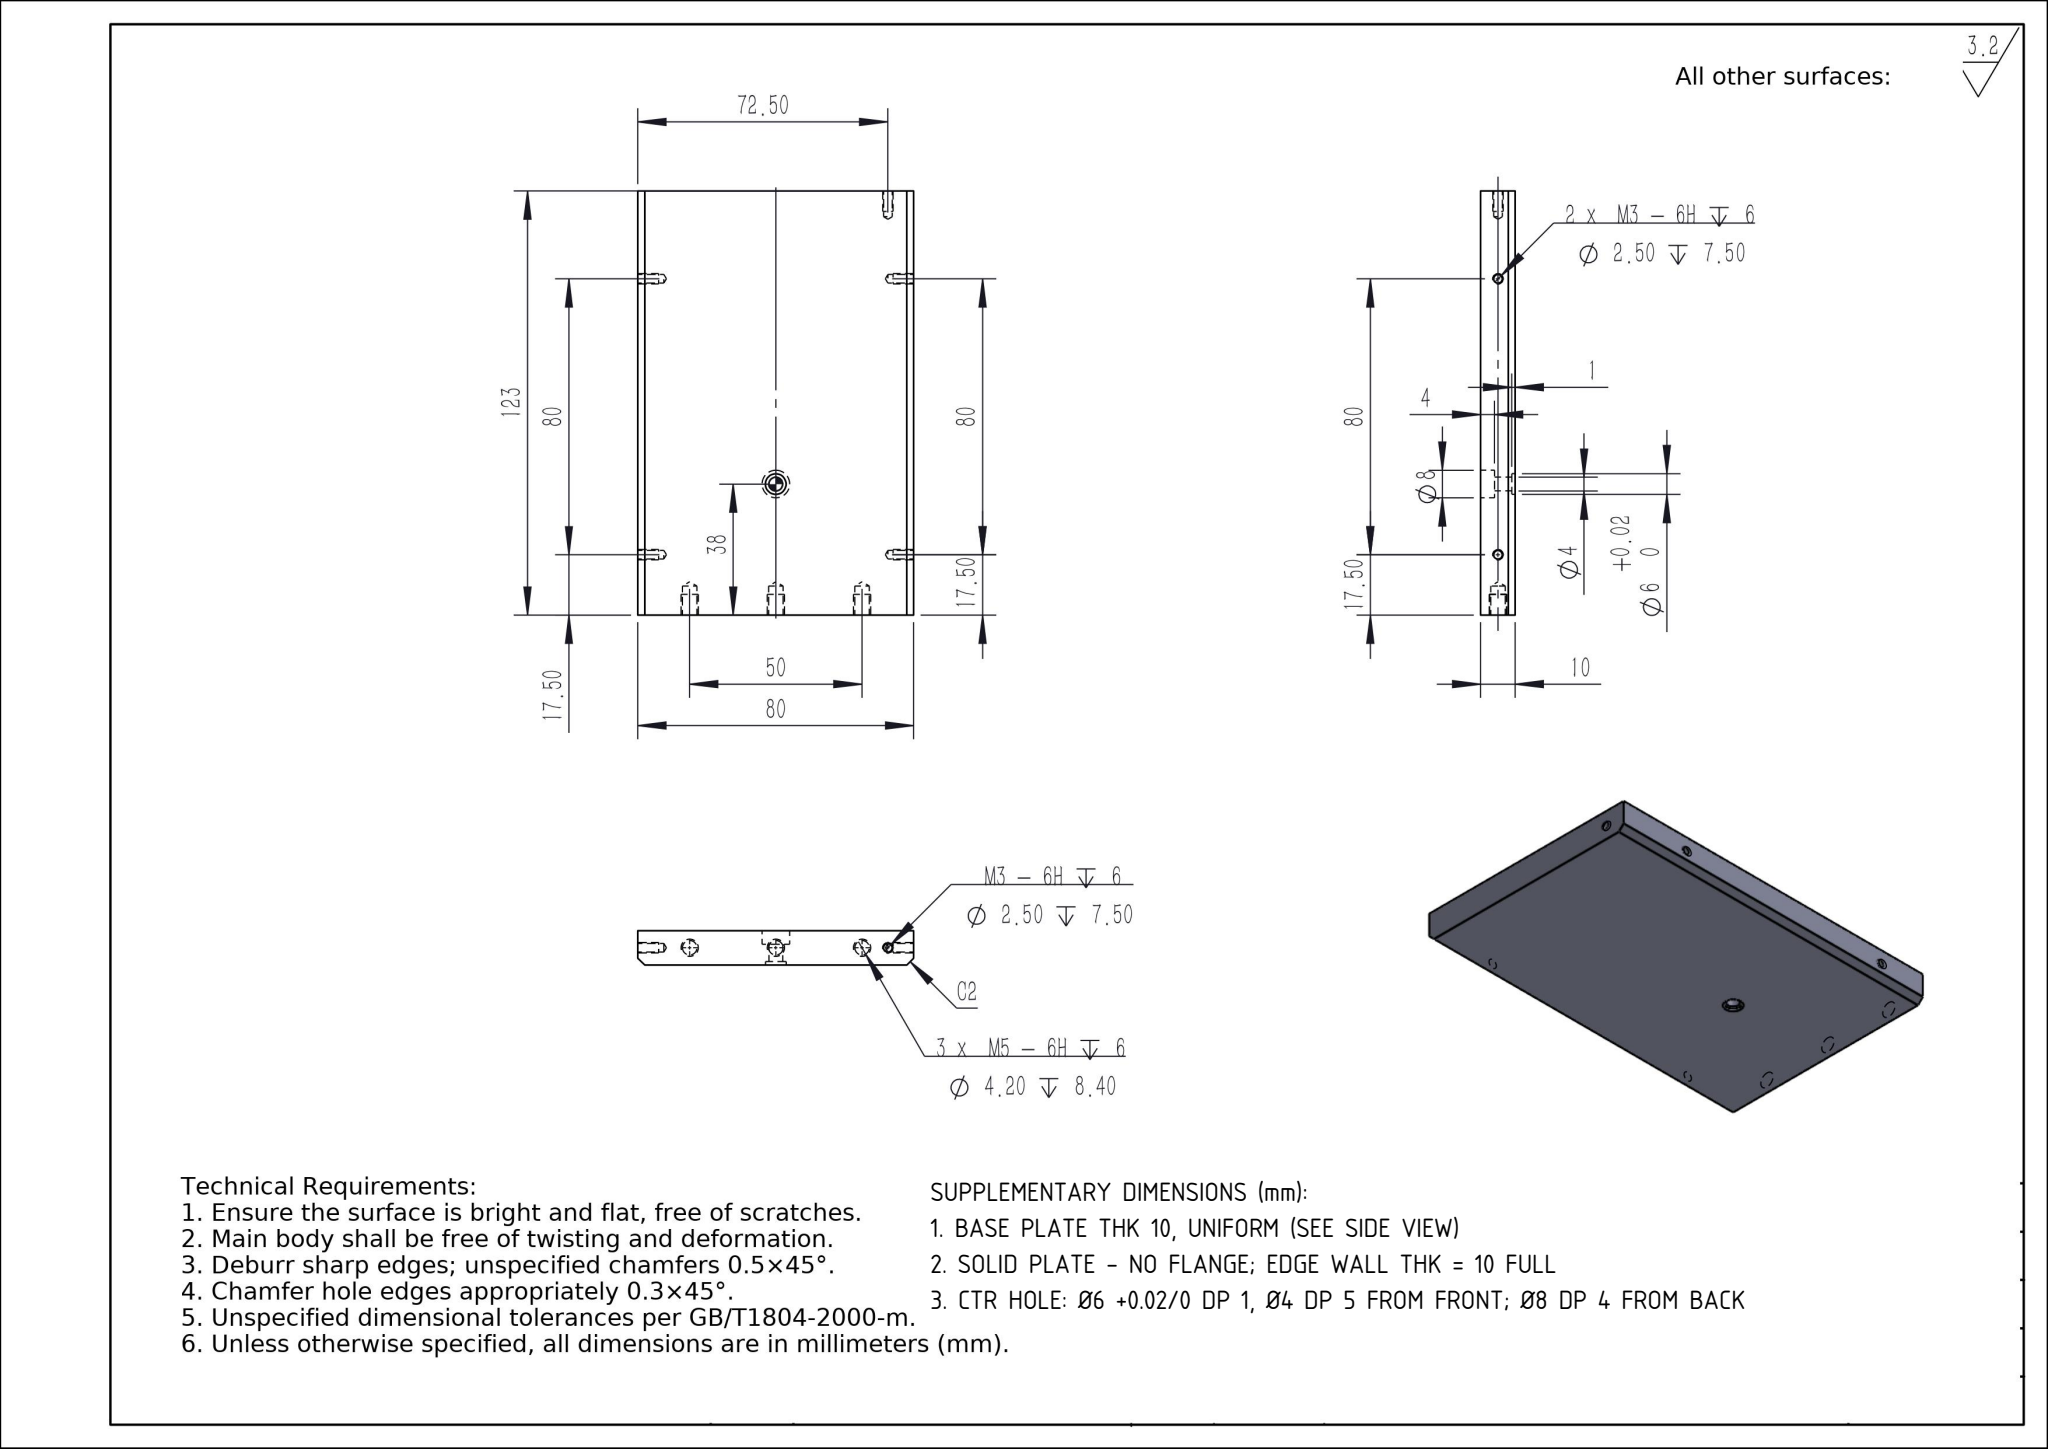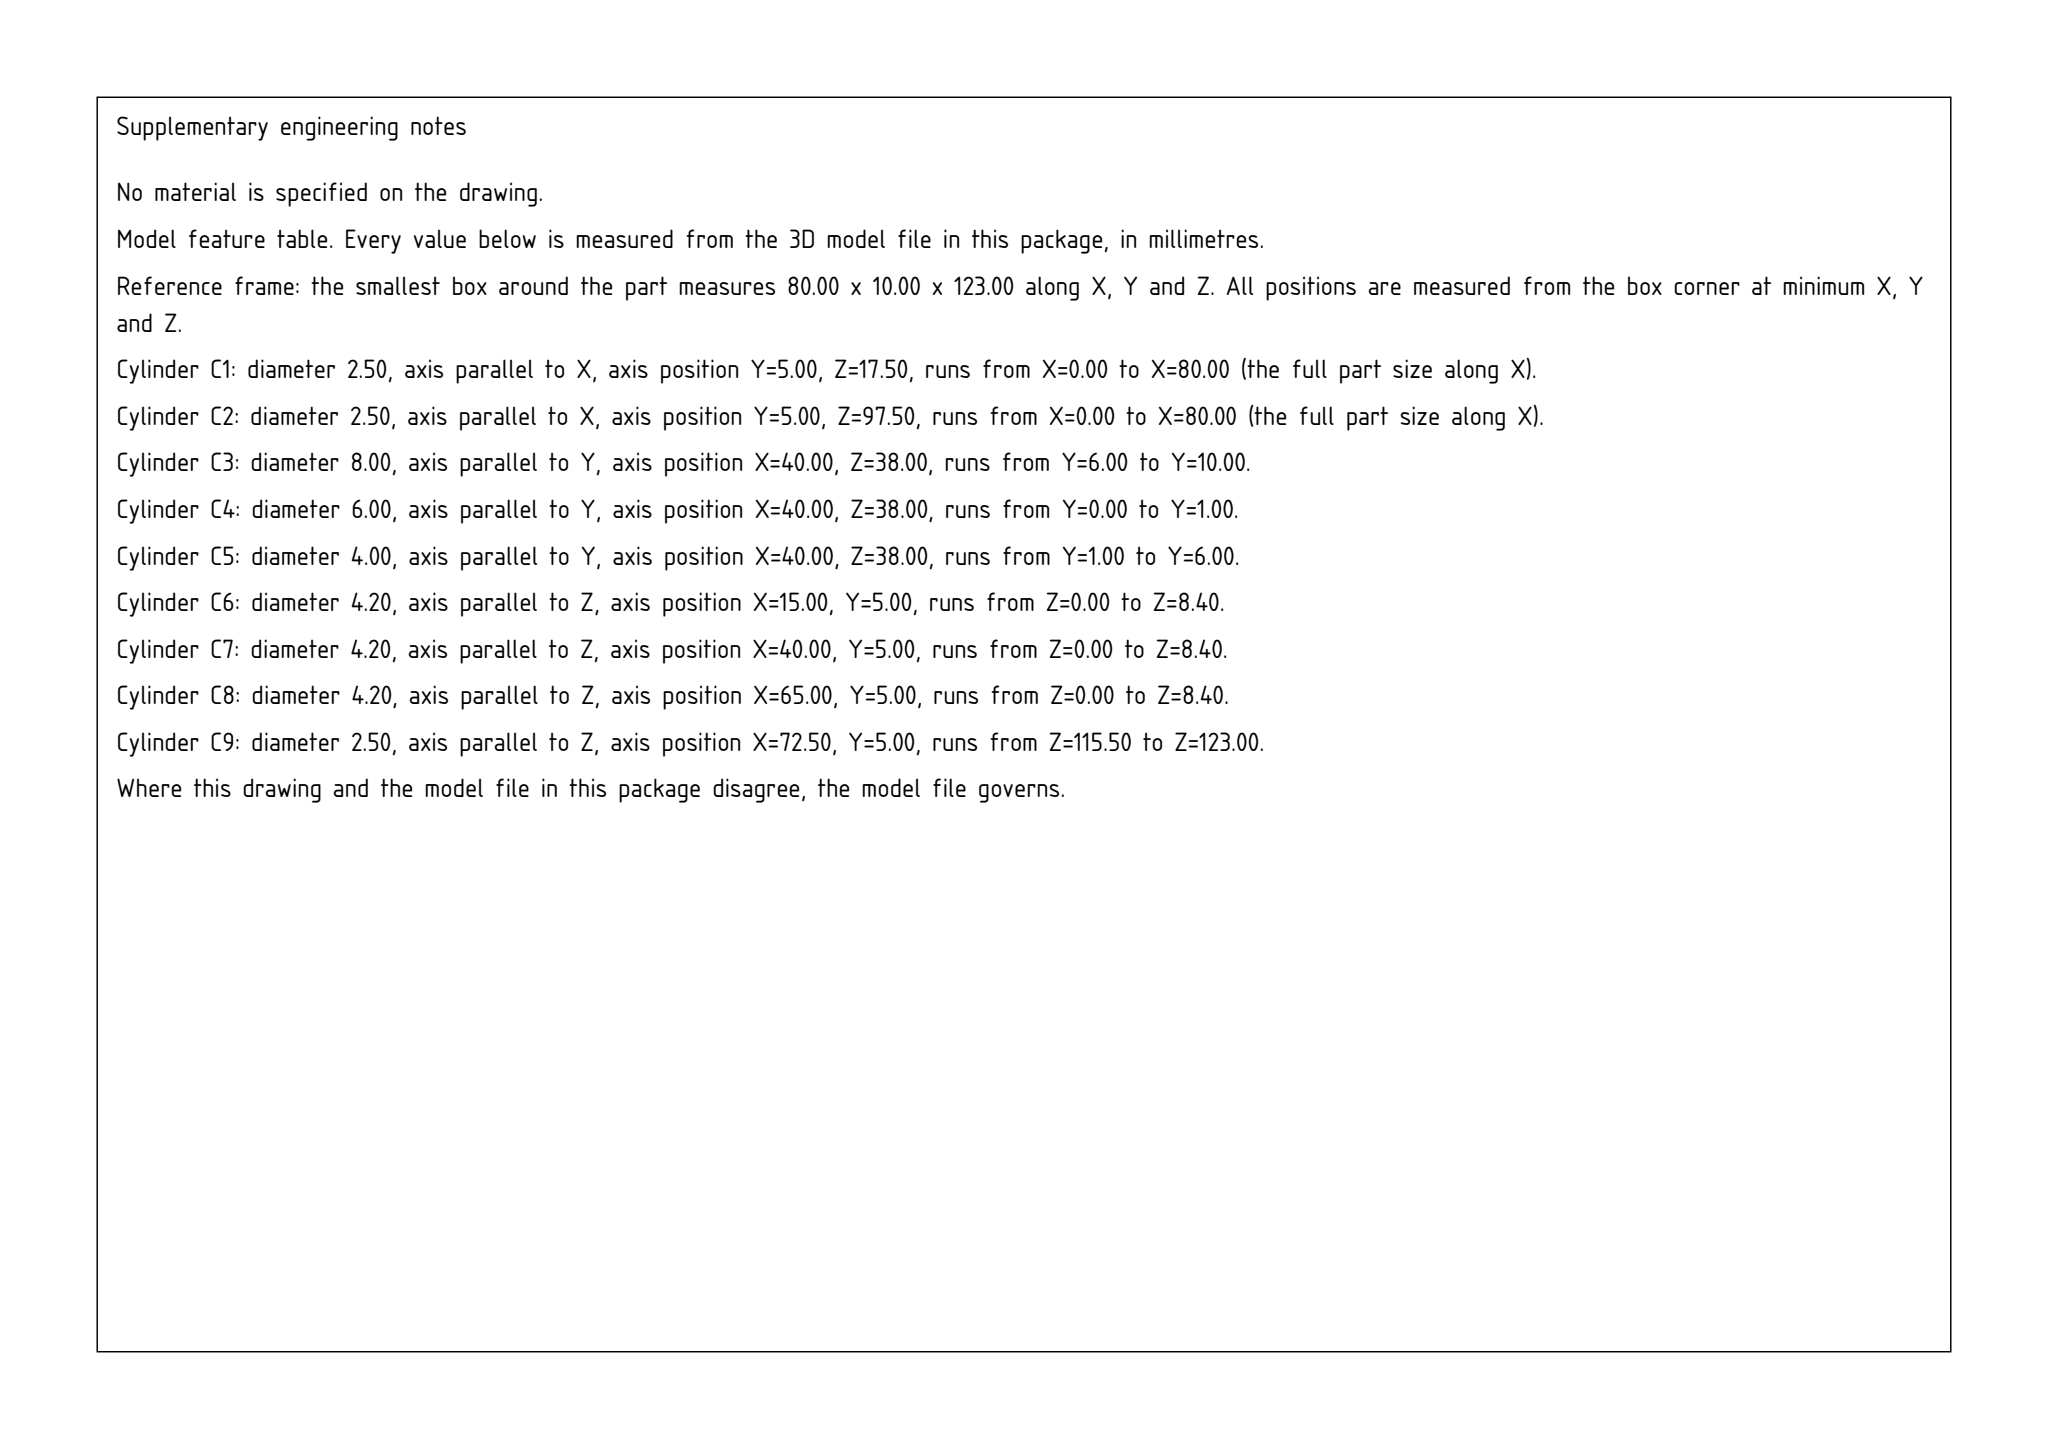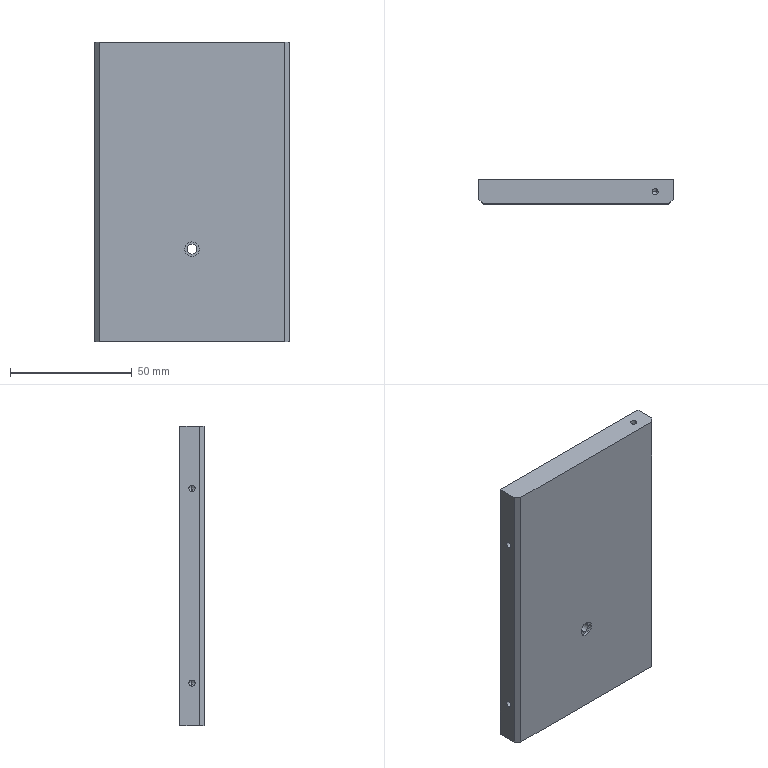Part | SolidWorks | mm | 1 solid | 48 faces | box 80 x 10 x 123 mm | volume 97059 mm3 | cylinder 22 | cone 16 | plane 10 | commonest cylinder face diameters 2.5 x10 4.2 x6 6 x2 8 x2 4 x2
build123d program:
from build123d import *

# Parameters (mm, degrees)
SKETCH1_W             = 80
SKETCH1_H             = 123
BOSS_EXTRUDE1_DEPTH   = 10
M5_TAPPED_HOLE1_D     = 4.2
M5_TAPPED_HOLE1_DEPTH = 8.4
M5_TAPPED_HOLE1_TIP   = 1.262
CHAMFER1_SIZE         = 2
M3_TAPPED_HOLE1_D     = 4
SKETCH6_R             = 4
CUT_EXTRUDE1_DEPTH    = 4
SKETCH8_R             = 3
CUT_EXTRUDE2_DEPTH    = 1
M3_TAPPED_HOLE2_D     = 2.5
M3_TAPPED_HOLE2_DEPTH = 7.5
M3_TAPPED_HOLE2_TIP   = 0.7511
M3_TAPPED_HOLE3_D     = 2.5
M3_TAPPED_HOLE3_DEPTH = 7.5
M3_TAPPED_HOLE3_TIP   = 0.7511
M3_TAPPED_HOLE4_D     = 2.5
M3_TAPPED_HOLE4_DEPTH = 7.5
M3_TAPPED_HOLE4_TIP   = 0.7511


with BuildPart() as part:
    # Sketch1 → Boss-Extrude1 (new body)
    with BuildSketch(Plane(origin=(0, 0, 0), x_dir=(1, 0, 0), z_dir=(0, 1, 0))):
        Rectangle(SKETCH1_W, SKETCH1_H)
    extrude(amount=BOSS_EXTRUDE1_DEPTH)

    # M5 Tapped Hole1
    with Locations(Plane(origin=(0, 0, -61.5), x_dir=(-1, 0, 0), z_dir=(0, 0, -1))):
        with Locations((-25, 5), (25, 5), (0, 5)):
            Hole(M5_TAPPED_HOLE1_D / 2, depth=M5_TAPPED_HOLE1_DEPTH)
            with Locations((0, 0, -(M5_TAPPED_HOLE1_DEPTH + M5_TAPPED_HOLE1_TIP / 2))):  # 118° drill point
                Cone(0, M5_TAPPED_HOLE1_D / 2, M5_TAPPED_HOLE1_TIP, mode=Mode.SUBTRACT)

    # Chamfer1
    chamfer1_edges = [part.edges().sort_by_distance(p)[0] for p in [
        (-40, 0, 0),
        (40, 0, 0),
    ]]
    chamfer(chamfer1_edges, length=CHAMFER1_SIZE)

    # M3 Tapped Hole1 (through all)
    with Locations(Plane(origin=(0, 0, 0), x_dir=(-1, 0, 0), z_dir=(0, -1, 0))):
        with Locations((0, 23.5)):
            Hole(M3_TAPPED_HOLE1_D / 2)

    # Sketch6 → Cut-Extrude1 (cut)
    with BuildSketch(Plane(origin=(0, 10, 0), x_dir=(1, 0, 0), z_dir=(0, 1, 0))):
        with Locations(Location((0, 23.5, 0), (0, 0, 270))):
            Circle(SKETCH6_R)
    extrude(amount=-CUT_EXTRUDE1_DEPTH, mode=Mode.SUBTRACT)

    # Sketch8 → Cut-Extrude2 (cut)
    with BuildSketch(Plane.XZ):
        with Locations(Location((0, -23.5, 0), (0, 0, 270))):
            Circle(SKETCH8_R)
    extrude(amount=-CUT_EXTRUDE2_DEPTH, mode=Mode.SUBTRACT)

    # M3 Tapped Hole2
    with Locations(Plane(origin=(40, 0, 0), x_dir=(0, 0, -1), z_dir=(1, 0, 0))):
        with Locations((44, 5), (-36, 5)):
            Hole(M3_TAPPED_HOLE2_D / 2, depth=M3_TAPPED_HOLE2_DEPTH)
            with Locations((0, 0, -(M3_TAPPED_HOLE2_DEPTH + M3_TAPPED_HOLE2_TIP / 2))):  # 118° drill point
                Cone(0, M3_TAPPED_HOLE2_D / 2, M3_TAPPED_HOLE2_TIP, mode=Mode.SUBTRACT)

    # M3 Tapped Hole3
    with Locations(Plane.XY.offset(61.5)):
        with Locations((32.5, 5)):
            Hole(M3_TAPPED_HOLE3_D / 2, depth=M3_TAPPED_HOLE3_DEPTH)
            with Locations((0, 0, -(M3_TAPPED_HOLE3_DEPTH + M3_TAPPED_HOLE3_TIP / 2))):  # 118° drill point
                Cone(0, M3_TAPPED_HOLE3_D / 2, M3_TAPPED_HOLE3_TIP, mode=Mode.SUBTRACT)

    # M3 Tapped Hole4
    with Locations(Plane.ZY.offset(40)):
        with Locations((36, 5), (-44, 5)):
            Hole(M3_TAPPED_HOLE4_D / 2, depth=M3_TAPPED_HOLE4_DEPTH)
            with Locations((0, 0, -(M3_TAPPED_HOLE4_DEPTH + M3_TAPPED_HOLE4_TIP / 2))):  # 118° drill point
                Cone(0, M3_TAPPED_HOLE4_D / 2, M3_TAPPED_HOLE4_TIP, mode=Mode.SUBTRACT)


solid = part.part